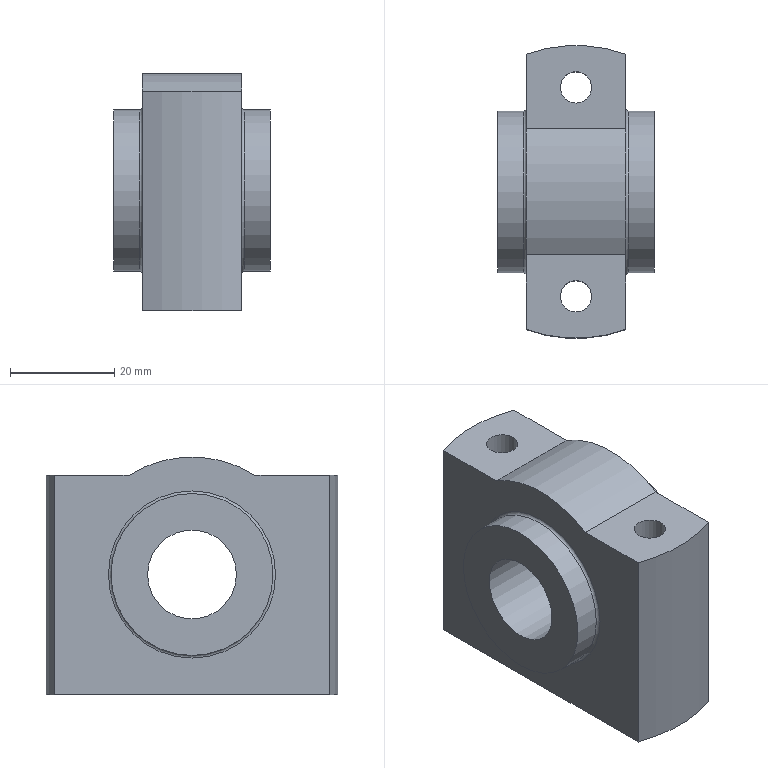Component | NX | FLYWHEEL_SUPPORT_FRAME | 1 solid | 17 faces | volume 44030 mm3 | cylinder 8 | plane 7 | torus 2 | commonest cylinder face diameters 56 x2 31 x2 6 x2 45 x1 17 x1